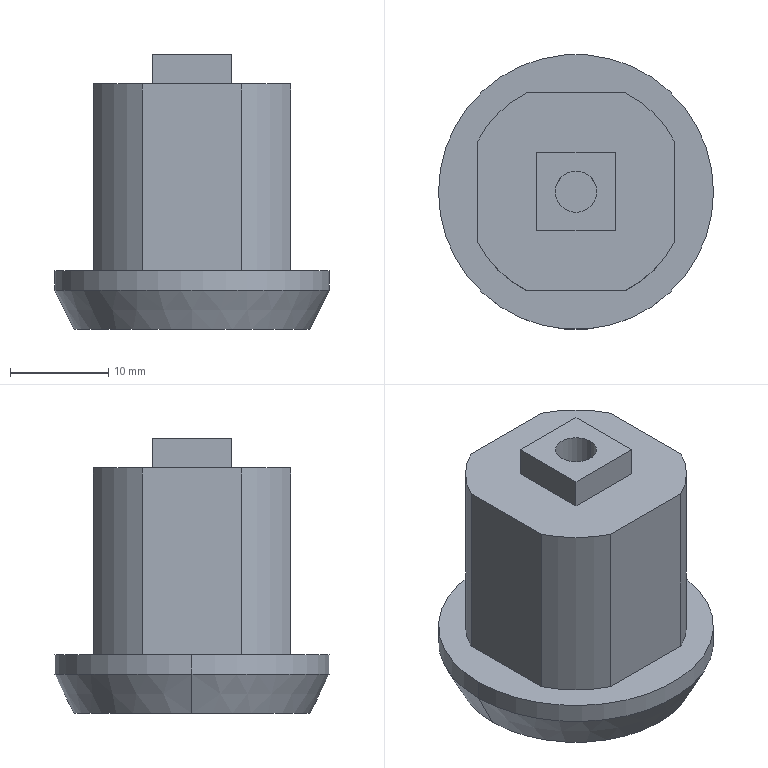Component | SolidWorks | LeftDoorPanelAssembly-1_Lock(MS407)-1 | 1 solid | 32 faces | box 28 x 28 x 28 mm | volume 10078 mm3 | plane 22 | cylinder 8 | cone 2 | commonest cylinder face diameters 22.5 x4 4.2 x2 28 x2
build123d program:
from build123d import *

# Parameters (mm, degrees)
BOSS_EXTRUDE1_DEPTH = 19
SKETCH2_R           = 14
BOSS_EXTRUDE2_DEPTH = 6
CHAMFER1_SIZE       = 4
CHAMFER1_SIZE2      = 2
SKETCH3_W           = 2.8
SKETCH3_H           = 12
CUT_EXTRUDE1_DEPTH  = 10
SKETCH4_W           = 8
SKETCH4_H           = 8
BOSS_EXTRUDE3_DEPTH = 3
SKETCH5_R           = 2.1
CUT_EXTRUDE2_DEPTH  = 5
CHAMFER2_SIZE       = 0.2


with BuildPart() as part:
    # Sketch1 → Boss-Extrude1 (new body)
    with BuildSketch(Plane.XY):
        with BuildLine():
            Line((-10.05, 5.056), (-10.05, -5.056))
            ThreePointArc((-10.05, -5.056), (-7.955, -7.955), (-5.056, -10.05))
            Line((-5.056, -10.05), (5.056, -10.05))
            ThreePointArc((5.056, -10.05), (7.955, -7.955), (10.05, -5.056))
            Line((10.05, -5.056), (10.05, 5.056))
            ThreePointArc((10.05, 5.056), (7.955, 7.955), (5.056, 10.05))
            Line((5.056, 10.05), (-5.056, 10.05))
            ThreePointArc((-5.056, 10.05), (-7.955, 7.955), (-10.05, 5.056))
        make_face()
    extrude(amount=BOSS_EXTRUDE1_DEPTH)

    # Sketch2 → Boss-Extrude2 (add)
    with BuildSketch(Plane(origin=(0, 0, 0), x_dir=(-1, 0, 0), z_dir=(0, 0, -1))):
        Circle(SKETCH2_R)
    extrude(amount=BOSS_EXTRUDE2_DEPTH)

    # Chamfer1
    chamfer1_edges = [part.edges().sort_by_distance(p)[0] for p in [
        (14, 0, -6),
    ]]
    chamfer1_side = [part.faces().sort_by_distance(p)[0] for p in [
        (14, 0, -3),
    ]]
    chamfer(chamfer1_edges, length=CHAMFER1_SIZE, length2=CHAMFER1_SIZE2, reference=chamfer1_side[0])

    # Sketch3 → Cut-Extrude1 (cut)
    with BuildSketch(Plane(origin=(0, 0, -6), x_dir=(-1, 0, 0), z_dir=(0, 0, -1))):
        Rectangle(SKETCH3_W, SKETCH3_H)
    extrude(amount=-CUT_EXTRUDE1_DEPTH, mode=Mode.SUBTRACT)

    # Sketch4 → Boss-Extrude3 (add)
    with BuildSketch(Plane.XY.offset(19)):
        Rectangle(SKETCH4_W, SKETCH4_H)
    extrude(amount=BOSS_EXTRUDE3_DEPTH)

    # Sketch5 → Cut-Extrude2 (cut)
    with BuildSketch(Plane.XY.offset(22)):
        Circle(SKETCH5_R)
    extrude(amount=-CUT_EXTRUDE2_DEPTH, mode=Mode.SUBTRACT)

    # Chamfer2
    chamfer2_edges = [part.edges().sort_by_distance(p)[0] for p in [
        (1.4, 0, -6),
        (0, -6, -6),
        (-1.4, 0, -6),
        (0, 6, -6),
    ]]
    chamfer(chamfer2_edges, length=CHAMFER2_SIZE)


solid = part.part

# Placed as in the assembly
solid = solid.moved(Location((0.6118, 13.542, -73.1), (0, 0, 0)))
STEP:
#1=CARTESIAN_POINT('',(-0.05859,0.5331,-2.209));
#2=VERTEX_POINT('',#1);
#3=CARTESIAN_POINT('',(0.1068,0.5331,-2.209));
#4=VERTEX_POINT('',#3);
#5=CARTESIAN_POINT('',(0.02409,0.5331,-2.209));
#6=DIRECTION('',(0.,0.,1.));
#7=DIRECTION('',(1.,0.,0.));
#8=AXIS2_PLACEMENT_3D('',#5,#6,#7);
#9=CIRCLE('',#8,0.08268);
#10=EDGE_CURVE('',#2,#4,#9,.T.);
#11=ORIENTED_EDGE('',*,*,#10,.F.);
#12=CARTESIAN_POINT('',(-0.05859,0.5331,-2.012));
#13=VERTEX_POINT('',#12);
#14=CARTESIAN_POINT('',(-0.05859,0.5331,-2.209));
#15=DIRECTION('',(0.,0.,1.));
#16=VECTOR('',#15,39.37);
#17=LINE('',#14,#16);
#18=EDGE_CURVE('',#2,#13,#17,.T.);
#19=ORIENTED_EDGE('',*,*,#18,.T.);
#20=CARTESIAN_POINT('',(0.1068,0.5331,-2.012));
#21=VERTEX_POINT('',#20);
#22=CARTESIAN_POINT('',(0.02409,0.5331,-2.012));
#23=DIRECTION('',(0.,0.,1.));
#24=DIRECTION('',(1.,0.,0.));
#25=AXIS2_PLACEMENT_3D('',#22,#23,#24);
#26=CIRCLE('',#25,0.08268);
#27=EDGE_CURVE('',#13,#21,#26,.T.);
#28=ORIENTED_EDGE('',*,*,#27,.T.);
#29=CARTESIAN_POINT('',(0.1068,0.5331,-2.209));
#30=DIRECTION('',(0.,0.,1.));
#31=VECTOR('',#30,39.37);
#32=LINE('',#29,#31);
#33=EDGE_CURVE('',#4,#21,#32,.T.);
#34=ORIENTED_EDGE('',*,*,#33,.F.);
#35=EDGE_LOOP('',(#11,#19,#28,#34));
#36=FACE_OUTER_BOUND('',#35,.T.);
#37=CARTESIAN_POINT('',(0.02409,0.5331,-2.209));
#38=DIRECTION('',(0.,0.,1.));
#39=DIRECTION('',(1.,0.,0.));
#40=AXIS2_PLACEMENT_3D('',#37,#38,#39);
#41=CYLINDRICAL_SURFACE('',#40,0.08268);
#42=ADVANCED_FACE('',(#36),#41,.F.);
#43=CARTESIAN_POINT('',(-0.4484,0.5331,-3.114));
#44=VERTEX_POINT('',#43);
#45=CARTESIAN_POINT('',(0.4965,0.5331,-3.114));
#46=VERTEX_POINT('',#45);
#47=CARTESIAN_POINT('',(0.02409,0.5331,-3.114));
#48=DIRECTION('',(0.,0.,-1.));
#49=DIRECTION('',(-1.,0.,0.));
#50=AXIS2_PLACEMENT_3D('',#47,#48,#49);
#51=CIRCLE('',#50,0.4724);
#52=EDGE_CURVE('',#44,#46,#51,.T.);
#53=ORIENTED_EDGE('',*,*,#52,.F.);
#54=CARTESIAN_POINT('',(-0.5271,0.5331,-2.957));
#55=VERTEX_POINT('',#54);
#56=CARTESIAN_POINT('',(-0.4484,0.5331,-3.114));
#57=DIRECTION('',(-0.4472,0.,0.8944));
#58=VECTOR('',#57,39.37);
#59=LINE('',#56,#58);
#60=EDGE_CURVE('',#44,#55,#59,.T.);
#61=ORIENTED_EDGE('',*,*,#60,.T.);
#62=CARTESIAN_POINT('',(0.5753,0.5331,-2.957));
#63=VERTEX_POINT('',#62);
#64=CARTESIAN_POINT('',(0.02409,0.5331,-2.957));
#65=DIRECTION('',(0.,0.,1.));
#66=DIRECTION('',(-1.,0.,0.));
#67=AXIS2_PLACEMENT_3D('',#64,#65,#66);
#68=CIRCLE('',#67,0.5512);
#69=EDGE_CURVE('',#63,#55,#68,.T.);
#70=ORIENTED_EDGE('',*,*,#69,.F.);
#71=CARTESIAN_POINT('',(0.4965,0.5331,-3.114));
#72=DIRECTION('',(0.4472,0.,0.8944));
#73=VECTOR('',#72,39.37);
#74=LINE('',#71,#73);
#75=EDGE_CURVE('',#46,#63,#74,.T.);
#76=ORIENTED_EDGE('',*,*,#75,.F.);
#77=EDGE_LOOP('',(#53,#61,#70,#76));
#78=FACE_OUTER_BOUND('',#77,.T.);
#79=CARTESIAN_POINT('',(0.02409,0.5331,-3.114));
#80=DIRECTION('',(0.,0.,1.));
#81=DIRECTION('',(1.,0.,0.));
#82=AXIS2_PLACEMENT_3D('',#79,#80,#81);
#83=CONICAL_SURFACE('',#82,0.4724,0.4636);
#84=ADVANCED_FACE('',(#78),#83,.T.);
#85=ORIENTED_EDGE('',*,*,#69,.T.);
#86=CARTESIAN_POINT('',(-0.5271,0.5331,-2.878));
#87=VERTEX_POINT('',#86);
#88=CARTESIAN_POINT('',(-0.5271,0.5331,-3.114));
#89=DIRECTION('',(0.,0.,1.));
#90=VECTOR('',#89,39.37);
#91=LINE('',#88,#90);
#92=EDGE_CURVE('',#55,#87,#91,.T.);
#93=ORIENTED_EDGE('',*,*,#92,.T.);
#94=CARTESIAN_POINT('',(0.5753,0.5331,-2.878));
#95=VERTEX_POINT('',#94);
#96=CARTESIAN_POINT('',(0.02409,0.5331,-2.878));
#97=DIRECTION('',(0.,0.,-1.));
#98=DIRECTION('',(-1.,0.,0.));
#99=AXIS2_PLACEMENT_3D('',#96,#97,#98);
#100=CIRCLE('',#99,0.5512);
#101=EDGE_CURVE('',#87,#95,#100,.T.);
#102=ORIENTED_EDGE('',*,*,#101,.T.);
#103=CARTESIAN_POINT('',(0.5753,0.5331,-3.114));
#104=DIRECTION('',(0.,0.,1.));
#105=VECTOR('',#104,39.37);
#106=LINE('',#103,#105);
#107=EDGE_CURVE('',#63,#95,#106,.T.);
#108=ORIENTED_EDGE('',*,*,#107,.F.);
#109=EDGE_LOOP('',(#85,#93,#102,#108));
#110=FACE_OUTER_BOUND('',#109,.T.);
#111=CARTESIAN_POINT('',(0.02409,0.5331,-3.114));
#112=DIRECTION('',(0.,0.,1.));
#113=DIRECTION('',(1.,0.,0.));
#114=AXIS2_PLACEMENT_3D('',#111,#112,#113);
#115=CYLINDRICAL_SURFACE('',#114,0.5512);
#116=ADVANCED_FACE('',(#110),#115,.T.);
#117=CARTESIAN_POINT('',(-0.175,0.9288,-2.13));
#118=VERTEX_POINT('',#117);
#119=CARTESIAN_POINT('',(-0.3716,0.7322,-2.13));
#120=VERTEX_POINT('',#119);
#121=CARTESIAN_POINT('',(0.02409,0.5331,-2.13));
#122=DIRECTION('',(0.,0.,1.));
#123=DIRECTION('',(1.,0.,0.));
#124=AXIS2_PLACEMENT_3D('',#121,#122,#123);
#125=CIRCLE('',#124,0.4429);
#126=EDGE_CURVE('',#118,#120,#125,.T.);
#127=ORIENTED_EDGE('',*,*,#126,.T.);
#128=CARTESIAN_POINT('',(-0.3716,0.3341,-2.13));
#129=VERTEX_POINT('',#128);
#130=CARTESIAN_POINT('',(-0.3716,0.7322,-2.13));
#131=DIRECTION('',(0.,-1.,0.));
#132=VECTOR('',#131,39.37);
#133=LINE('',#130,#132);
#134=EDGE_CURVE('',#120,#129,#133,.T.);
#135=ORIENTED_EDGE('',*,*,#134,.T.);
#136=CARTESIAN_POINT('',(-0.175,0.1375,-2.13));
#137=VERTEX_POINT('',#136);
#138=CARTESIAN_POINT('',(0.02409,0.5331,-2.13));
#139=DIRECTION('',(0.,0.,1.));
#140=DIRECTION('',(1.,0.,0.));
#141=AXIS2_PLACEMENT_3D('',#138,#139,#140);
#142=CIRCLE('',#141,0.4429);
#143=EDGE_CURVE('',#129,#137,#142,.T.);
#144=ORIENTED_EDGE('',*,*,#143,.T.);
#145=CARTESIAN_POINT('',(0.2231,0.1375,-2.13));
#146=VERTEX_POINT('',#145);
#147=CARTESIAN_POINT('',(-0.175,0.1375,-2.13));
#148=DIRECTION('',(1.,0.,0.));
#149=VECTOR('',#148,39.37);
#150=LINE('',#147,#149);
#151=EDGE_CURVE('',#137,#146,#150,.T.);
#152=ORIENTED_EDGE('',*,*,#151,.T.);
#153=CARTESIAN_POINT('',(0.4198,0.3341,-2.13));
#154=VERTEX_POINT('',#153);
#155=CARTESIAN_POINT('',(0.02409,0.5331,-2.13));
#156=DIRECTION('',(0.,0.,1.));
#157=DIRECTION('',(1.,0.,0.));
#158=AXIS2_PLACEMENT_3D('',#155,#156,#157);
#159=CIRCLE('',#158,0.4429);
#160=EDGE_CURVE('',#146,#154,#159,.T.);
#161=ORIENTED_EDGE('',*,*,#160,.T.);
#162=CARTESIAN_POINT('',(0.4198,0.7322,-2.13));
#163=VERTEX_POINT('',#162);
#164=CARTESIAN_POINT('',(0.4198,0.3341,-2.13));
#165=DIRECTION('',(0.,1.,0.));
#166=VECTOR('',#165,39.37);
#167=LINE('',#164,#166);
#168=EDGE_CURVE('',#154,#163,#167,.T.);
#169=ORIENTED_EDGE('',*,*,#168,.T.);
#170=CARTESIAN_POINT('',(0.2231,0.9288,-2.13));
#171=VERTEX_POINT('',#170);
#172=CARTESIAN_POINT('',(0.02409,0.5331,-2.13));
#173=DIRECTION('',(0.,0.,1.));
#174=DIRECTION('',(1.,0.,0.));
#175=AXIS2_PLACEMENT_3D('',#172,#173,#174);
#176=CIRCLE('',#175,0.4429);
#177=EDGE_CURVE('',#163,#171,#176,.T.);
#178=ORIENTED_EDGE('',*,*,#177,.T.);
#179=CARTESIAN_POINT('',(0.2231,0.9288,-2.13));
#180=DIRECTION('',(-1.,0.,0.));
#181=VECTOR('',#180,39.37);
#182=LINE('',#179,#181);
#183=EDGE_CURVE('',#171,#118,#182,.T.);
#184=ORIENTED_EDGE('',*,*,#183,.T.);
#185=EDGE_LOOP('',(#127,#135,#144,#152,#161,#169,#178,#184));
#186=FACE_OUTER_BOUND('',#185,.T.);
#187=CARTESIAN_POINT('',(-0.1334,0.3757,-2.13));
#188=VERTEX_POINT('',#187);
#189=CARTESIAN_POINT('',(0.1816,0.3757,-2.13));
#190=VERTEX_POINT('',#189);
#191=CARTESIAN_POINT('',(0.1816,0.3757,-2.13));
#192=DIRECTION('',(1.,0.,0.));
#193=VECTOR('',#192,39.37);
#194=LINE('',#191,#193);
#195=EDGE_CURVE('',#188,#190,#194,.T.);
#196=ORIENTED_EDGE('',*,*,#195,.F.);
#197=CARTESIAN_POINT('',(-0.1334,0.6906,-2.13));
#198=VERTEX_POINT('',#197);
#199=CARTESIAN_POINT('',(-0.1334,0.3757,-2.13));
#200=DIRECTION('',(0.,-1.,0.));
#201=VECTOR('',#200,39.37);
#202=LINE('',#199,#201);
#203=EDGE_CURVE('',#198,#188,#202,.T.);
#204=ORIENTED_EDGE('',*,*,#203,.F.);
#205=CARTESIAN_POINT('',(0.1816,0.6906,-2.13));
#206=VERTEX_POINT('',#205);
#207=CARTESIAN_POINT('',(0.1816,0.6906,-2.13));
#208=DIRECTION('',(-1.,-0.,0.));
#209=VECTOR('',#208,39.37);
#210=LINE('',#207,#209);
#211=EDGE_CURVE('',#206,#198,#210,.T.);
#212=ORIENTED_EDGE('',*,*,#211,.F.);
#213=CARTESIAN_POINT('',(0.1816,0.3757,-2.13));
#214=DIRECTION('',(0.,1.,0.));
#215=VECTOR('',#214,39.37);
#216=LINE('',#213,#215);
#217=EDGE_CURVE('',#190,#206,#216,.T.);
#218=ORIENTED_EDGE('',*,*,#217,.F.);
#219=EDGE_LOOP('',(#196,#204,#212,#218));
#220=FACE_BOUND('',#219,.T.);
#221=CARTESIAN_POINT('',(0.02409,0.5331,-2.13));
#222=DIRECTION('',(0.,0.,1.));
#223=DIRECTION('',(1.,0.,0.));
#224=AXIS2_PLACEMENT_3D('',#221,#222,#223);
#225=PLANE('',#224);
#226=ADVANCED_FACE('',(#186,#220),#225,.T.);
#227=CARTESIAN_POINT('',(-0.175,0.9288,-2.878));
#228=VERTEX_POINT('',#227);
#229=CARTESIAN_POINT('',(-0.3716,0.7322,-2.878));
#230=VERTEX_POINT('',#229);
#231=CARTESIAN_POINT('',(0.02409,0.5331,-2.878));
#232=DIRECTION('',(0.,0.,1.));
#233=DIRECTION('',(1.,0.,0.));
#234=AXIS2_PLACEMENT_3D('',#231,#232,#233);
#235=CIRCLE('',#234,0.4429);
#236=EDGE_CURVE('',#228,#230,#235,.T.);
#237=ORIENTED_EDGE('',*,*,#236,.T.);
#238=CARTESIAN_POINT('',(-0.3716,0.7322,-2.13));
#239=DIRECTION('',(0.,0.,-1.));
#240=VECTOR('',#239,39.37);
#241=LINE('',#238,#240);
#242=EDGE_CURVE('',#120,#230,#241,.T.);
#243=ORIENTED_EDGE('',*,*,#242,.F.);
#244=ORIENTED_EDGE('',*,*,#126,.F.);
#245=CARTESIAN_POINT('',(-0.175,0.9288,-2.13));
#246=DIRECTION('',(0.,0.,-1.));
#247=VECTOR('',#246,39.37);
#248=LINE('',#245,#247);
#249=EDGE_CURVE('',#118,#228,#248,.T.);
#250=ORIENTED_EDGE('',*,*,#249,.T.);
#251=EDGE_LOOP('',(#237,#243,#244,#250));
#252=FACE_OUTER_BOUND('',#251,.T.);
#253=CARTESIAN_POINT('',(0.02409,0.5331,-2.13));
#254=DIRECTION('',(0.,0.,-1.));
#255=DIRECTION('',(-1.,0.,0.));
#256=AXIS2_PLACEMENT_3D('',#253,#254,#255);
#257=CYLINDRICAL_SURFACE('',#256,0.4429);
#258=ADVANCED_FACE('',(#252),#257,.T.);
#259=CARTESIAN_POINT('',(-0.3716,0.3341,-2.878));
#260=VERTEX_POINT('',#259);
#261=CARTESIAN_POINT('',(-0.3716,0.7322,-2.878));
#262=DIRECTION('',(0.,-1.,0.));
#263=VECTOR('',#262,39.37);
#264=LINE('',#261,#263);
#265=EDGE_CURVE('',#230,#260,#264,.T.);
#266=ORIENTED_EDGE('',*,*,#265,.T.);
#267=CARTESIAN_POINT('',(-0.3716,0.3341,-2.13));
#268=DIRECTION('',(0.,0.,-1.));
#269=VECTOR('',#268,39.37);
#270=LINE('',#267,#269);
#271=EDGE_CURVE('',#129,#260,#270,.T.);
#272=ORIENTED_EDGE('',*,*,#271,.F.);
#273=ORIENTED_EDGE('',*,*,#134,.F.);
#274=ORIENTED_EDGE('',*,*,#242,.T.);
#275=EDGE_LOOP('',(#266,#272,#273,#274));
#276=FACE_OUTER_BOUND('',#275,.T.);
#277=CARTESIAN_POINT('',(-0.3716,0.7322,-2.13));
#278=DIRECTION('',(1.,0.,0.));
#279=DIRECTION('',(0.,0.,-1.));
#280=AXIS2_PLACEMENT_3D('',#277,#278,#279);
#281=PLANE('',#280);
#282=ADVANCED_FACE('',(#276),#281,.F.);
#283=CARTESIAN_POINT('',(-0.175,0.1375,-2.878));
#284=VERTEX_POINT('',#283);
#285=CARTESIAN_POINT('',(0.02409,0.5331,-2.878));
#286=DIRECTION('',(0.,0.,1.));
#287=DIRECTION('',(1.,0.,0.));
#288=AXIS2_PLACEMENT_3D('',#285,#286,#287);
#289=CIRCLE('',#288,0.4429);
#290=EDGE_CURVE('',#260,#284,#289,.T.);
#291=ORIENTED_EDGE('',*,*,#290,.T.);
#292=CARTESIAN_POINT('',(-0.175,0.1375,-2.13));
#293=DIRECTION('',(0.,0.,-1.));
#294=VECTOR('',#293,39.37);
#295=LINE('',#292,#294);
#296=EDGE_CURVE('',#137,#284,#295,.T.);
#297=ORIENTED_EDGE('',*,*,#296,.F.);
#298=ORIENTED_EDGE('',*,*,#143,.F.);
#299=ORIENTED_EDGE('',*,*,#271,.T.);
#300=EDGE_LOOP('',(#291,#297,#298,#299));
#301=FACE_OUTER_BOUND('',#300,.T.);
#302=CARTESIAN_POINT('',(0.02409,0.5331,-2.13));
#303=DIRECTION('',(0.,0.,-1.));
#304=DIRECTION('',(-1.,0.,0.));
#305=AXIS2_PLACEMENT_3D('',#302,#303,#304);
#306=CYLINDRICAL_SURFACE('',#305,0.4429);
#307=ADVANCED_FACE('',(#301),#306,.T.);
#308=CARTESIAN_POINT('',(0.2231,0.1375,-2.878));
#309=VERTEX_POINT('',#308);
#310=CARTESIAN_POINT('',(-0.175,0.1375,-2.878));
#311=DIRECTION('',(1.,0.,0.));
#312=VECTOR('',#311,39.37);
#313=LINE('',#310,#312);
#314=EDGE_CURVE('',#284,#309,#313,.T.);
#315=ORIENTED_EDGE('',*,*,#314,.T.);
#316=CARTESIAN_POINT('',(0.2231,0.1375,-2.13));
#317=DIRECTION('',(0.,0.,-1.));
#318=VECTOR('',#317,39.37);
#319=LINE('',#316,#318);
#320=EDGE_CURVE('',#146,#309,#319,.T.);
#321=ORIENTED_EDGE('',*,*,#320,.F.);
#322=ORIENTED_EDGE('',*,*,#151,.F.);
#323=ORIENTED_EDGE('',*,*,#296,.T.);
#324=EDGE_LOOP('',(#315,#321,#322,#323));
#325=FACE_OUTER_BOUND('',#324,.T.);
#326=CARTESIAN_POINT('',(-0.175,0.1375,-2.13));
#327=DIRECTION('',(0.,1.,0.));
#328=DIRECTION('',(0.,0.,1.));
#329=AXIS2_PLACEMENT_3D('',#326,#327,#328);
#330=PLANE('',#329);
#331=ADVANCED_FACE('',(#325),#330,.F.);
#332=CARTESIAN_POINT('',(0.4198,0.3341,-2.878));
#333=VERTEX_POINT('',#332);
#334=CARTESIAN_POINT('',(0.02409,0.5331,-2.878));
#335=DIRECTION('',(0.,0.,1.));
#336=DIRECTION('',(1.,0.,0.));
#337=AXIS2_PLACEMENT_3D('',#334,#335,#336);
#338=CIRCLE('',#337,0.4429);
#339=EDGE_CURVE('',#309,#333,#338,.T.);
#340=ORIENTED_EDGE('',*,*,#339,.T.);
#341=CARTESIAN_POINT('',(0.4198,0.3341,-2.13));
#342=DIRECTION('',(0.,0.,-1.));
#343=VECTOR('',#342,39.37);
#344=LINE('',#341,#343);
#345=EDGE_CURVE('',#154,#333,#344,.T.);
#346=ORIENTED_EDGE('',*,*,#345,.F.);
#347=ORIENTED_EDGE('',*,*,#160,.F.);
#348=ORIENTED_EDGE('',*,*,#320,.T.);
#349=EDGE_LOOP('',(#340,#346,#347,#348));
#350=FACE_OUTER_BOUND('',#349,.T.);
#351=CARTESIAN_POINT('',(0.02409,0.5331,-2.13));
#352=DIRECTION('',(0.,0.,-1.));
#353=DIRECTION('',(-1.,0.,0.));
#354=AXIS2_PLACEMENT_3D('',#351,#352,#353);
#355=CYLINDRICAL_SURFACE('',#354,0.4429);
#356=ADVANCED_FACE('',(#350),#355,.T.);
#357=CARTESIAN_POINT('',(0.4198,0.7322,-2.878));
#358=VERTEX_POINT('',#357);
#359=CARTESIAN_POINT('',(0.4198,0.3341,-2.878));
#360=DIRECTION('',(0.,1.,0.));
#361=VECTOR('',#360,39.37);
#362=LINE('',#359,#361);
#363=EDGE_CURVE('',#333,#358,#362,.T.);
#364=ORIENTED_EDGE('',*,*,#363,.T.);
#365=CARTESIAN_POINT('',(0.4198,0.7322,-2.13));
#366=DIRECTION('',(0.,0.,-1.));
#367=VECTOR('',#366,39.37);
#368=LINE('',#365,#367);
#369=EDGE_CURVE('',#163,#358,#368,.T.);
#370=ORIENTED_EDGE('',*,*,#369,.F.);
#371=ORIENTED_EDGE('',*,*,#168,.F.);
#372=ORIENTED_EDGE('',*,*,#345,.T.);
#373=EDGE_LOOP('',(#364,#370,#371,#372));
#374=FACE_OUTER_BOUND('',#373,.T.);
#375=CARTESIAN_POINT('',(0.4198,0.3341,-2.13));
#376=DIRECTION('',(-1.,0.,0.));
#377=DIRECTION('',(-0.,-1.,0.));
#378=AXIS2_PLACEMENT_3D('',#375,#376,#377);
#379=PLANE('',#378);
#380=ADVANCED_FACE('',(#374),#379,.F.);
#381=CARTESIAN_POINT('',(0.2231,0.9288,-2.878));
#382=VERTEX_POINT('',#381);
#383=CARTESIAN_POINT('',(0.02409,0.5331,-2.878));
#384=DIRECTION('',(0.,0.,1.));
#385=DIRECTION('',(1.,0.,0.));
#386=AXIS2_PLACEMENT_3D('',#383,#384,#385);
#387=CIRCLE('',#386,0.4429);
#388=EDGE_CURVE('',#358,#382,#387,.T.);
#389=ORIENTED_EDGE('',*,*,#388,.T.);
#390=CARTESIAN_POINT('',(0.2231,0.9288,-2.13));
#391=DIRECTION('',(0.,0.,-1.));
#392=VECTOR('',#391,39.37);
#393=LINE('',#390,#392);
#394=EDGE_CURVE('',#171,#382,#393,.T.);
#395=ORIENTED_EDGE('',*,*,#394,.F.);
#396=ORIENTED_EDGE('',*,*,#177,.F.);
#397=ORIENTED_EDGE('',*,*,#369,.T.);
#398=EDGE_LOOP('',(#389,#395,#396,#397));
#399=FACE_OUTER_BOUND('',#398,.T.);
#400=CARTESIAN_POINT('',(0.02409,0.5331,-2.13));
#401=DIRECTION('',(0.,0.,-1.));
#402=DIRECTION('',(-1.,0.,0.));
#403=AXIS2_PLACEMENT_3D('',#400,#401,#402);
#404=CYLINDRICAL_SURFACE('',#403,0.4429);
#405=ADVANCED_FACE('',(#399),#404,.T.);
#406=CARTESIAN_POINT('',(0.2231,0.9288,-2.878));
#407=DIRECTION('',(-1.,0.,0.));
#408=VECTOR('',#407,39.37);
#409=LINE('',#406,#408);
#410=EDGE_CURVE('',#382,#228,#409,.T.);
#411=ORIENTED_EDGE('',*,*,#410,.T.);
#412=ORIENTED_EDGE('',*,*,#249,.F.);
#413=ORIENTED_EDGE('',*,*,#183,.F.);
#414=ORIENTED_EDGE('',*,*,#394,.T.);
#415=EDGE_LOOP('',(#411,#412,#413,#414));
#416=FACE_OUTER_BOUND('',#415,.T.);
#417=CARTESIAN_POINT('',(0.2231,0.9288,-2.13));
#418=DIRECTION('',(0.,-1.,0.));
#419=DIRECTION('',(0.,0.,-1.));
#420=AXIS2_PLACEMENT_3D('',#417,#418,#419);
#421=PLANE('',#420);
#422=ADVANCED_FACE('',(#416),#421,.F.);
#423=CARTESIAN_POINT('',(0.02409,0.5331,-2.878));
#424=DIRECTION('',(0.,0.,-1.));
#425=DIRECTION('',(-1.,0.,0.));
#426=AXIS2_PLACEMENT_3D('',#423,#424,#425);
#427=CIRCLE('',#426,0.5512);
#428=EDGE_CURVE('',#95,#87,#427,.T.);
#429=ORIENTED_EDGE('',*,*,#428,.F.);
#430=ORIENTED_EDGE('',*,*,#101,.F.);
#431=EDGE_LOOP('',(#429,#430));
#432=FACE_OUTER_BOUND('',#431,.T.);
#433=ORIENTED_EDGE('',*,*,#265,.F.);
#434=ORIENTED_EDGE('',*,*,#236,.F.);
#435=ORIENTED_EDGE('',*,*,#410,.F.);
#436=ORIENTED_EDGE('',*,*,#388,.F.);
#437=ORIENTED_EDGE('',*,*,#363,.F.);
#438=ORIENTED_EDGE('',*,*,#339,.F.);
#439=ORIENTED_EDGE('',*,*,#314,.F.);
#440=ORIENTED_EDGE('',*,*,#290,.F.);
#441=EDGE_LOOP('',(#433,#434,#435,#436,#437,#438,#439,#440));
#442=FACE_BOUND('',#441,.T.);
#443=CARTESIAN_POINT('',(0.02409,0.5331,-2.878));
#444=DIRECTION('',(0.,0.,-1.));
#445=DIRECTION('',(-1.,0.,0.));
#446=AXIS2_PLACEMENT_3D('',#443,#444,#445);
#447=PLANE('',#446);
#448=ADVANCED_FACE('',(#432,#442),#447,.F.);
#449=ORIENTED_EDGE('',*,*,#92,.F.);
#450=CARTESIAN_POINT('',(0.02409,0.5331,-2.957));
#451=DIRECTION('',(0.,0.,1.));
#452=DIRECTION('',(-1.,0.,0.));
#453=AXIS2_PLACEMENT_3D('',#450,#451,#452);
#454=CIRCLE('',#453,0.5512);
#455=EDGE_CURVE('',#55,#63,#454,.T.);
#456=ORIENTED_EDGE('',*,*,#455,.T.);
#457=ORIENTED_EDGE('',*,*,#107,.T.);
#458=ORIENTED_EDGE('',*,*,#428,.T.);
#459=EDGE_LOOP('',(#449,#456,#457,#458));
#460=FACE_OUTER_BOUND('',#459,.T.);
#461=CARTESIAN_POINT('',(0.02409,0.5331,-3.114));
#462=DIRECTION('',(0.,0.,1.));
#463=DIRECTION('',(1.,0.,0.));
#464=AXIS2_PLACEMENT_3D('',#461,#462,#463);
#465=CYLINDRICAL_SURFACE('',#464,0.5512);
#466=ADVANCED_FACE('',(#460),#465,.T.);
#467=CARTESIAN_POINT('',(-0.03891,0.289,-3.114));
#468=VERTEX_POINT('',#467);
#469=CARTESIAN_POINT('',(0.08708,0.289,-3.114));
#470=VERTEX_POINT('',#469);
#471=CARTESIAN_POINT('',(0.0792,0.289,-3.114));
#472=DIRECTION('',(1.,0.,0.));
#473=VECTOR('',#472,39.37);
#474=LINE('',#471,#473);
#475=EDGE_CURVE('',#468,#470,#474,.T.);
#476=ORIENTED_EDGE('',*,*,#475,.T.);
#477=CARTESIAN_POINT('',(0.08708,0.7772,-3.114));
#478=VERTEX_POINT('',#477);
#479=CARTESIAN_POINT('',(0.08708,0.7694,-3.114));
#480=DIRECTION('',(0.,1.,0.));
#481=VECTOR('',#480,39.37);
#482=LINE('',#479,#481);
#483=EDGE_CURVE('',#470,#478,#482,.T.);
#484=ORIENTED_EDGE('',*,*,#483,.T.);
#485=CARTESIAN_POINT('',(-0.03891,0.7772,-3.114));
#486=VERTEX_POINT('',#485);
#487=CARTESIAN_POINT('',(-0.03103,0.7772,-3.114));
#488=DIRECTION('',(-1.,0.,0.));
#489=VECTOR('',#488,39.37);
#490=LINE('',#487,#489);
#491=EDGE_CURVE('',#478,#486,#490,.T.);
#492=ORIENTED_EDGE('',*,*,#491,.T.);
#493=CARTESIAN_POINT('',(-0.03891,0.2969,-3.114));
#494=DIRECTION('',(0.,-1.,0.));
#495=VECTOR('',#494,39.37);
#496=LINE('',#493,#495);
#497=EDGE_CURVE('',#486,#468,#496,.T.);
#498=ORIENTED_EDGE('',*,*,#497,.T.);
#499=EDGE_LOOP('',(#476,#484,#492,#498));
#500=FACE_BOUND('',#499,.T.);
#501=CARTESIAN_POINT('',(0.02409,0.5331,-3.114));
#502=DIRECTION('',(0.,0.,-1.));
#503=DIRECTION('',(-1.,0.,0.));
#504=AXIS2_PLACEMENT_3D('',#501,#502,#503);
#505=CIRCLE('',#504,0.4724);
#506=EDGE_CURVE('',#46,#44,#505,.T.);
#507=ORIENTED_EDGE('',*,*,#506,.T.);
#508=ORIENTED_EDGE('',*,*,#52,.T.);
#509=EDGE_LOOP('',(#507,#508));
#510=FACE_OUTER_BOUND('',#509,.T.);
#511=CARTESIAN_POINT('',(0.02409,0.5331,-3.114));
#512=DIRECTION('',(0.,0.,-1.));
#513=DIRECTION('',(-1.,0.,0.));
#514=AXIS2_PLACEMENT_3D('',#511,#512,#513);
#515=PLANE('',#514);
#516=ADVANCED_FACE('',(#500,#510),#515,.T.);
#517=ORIENTED_EDGE('',*,*,#60,.F.);
#518=ORIENTED_EDGE('',*,*,#506,.F.);
#519=ORIENTED_EDGE('',*,*,#75,.T.);
#520=ORIENTED_EDGE('',*,*,#455,.F.);
#521=EDGE_LOOP('',(#517,#518,#519,#520));
#522=FACE_OUTER_BOUND('',#521,.T.);
#523=CARTESIAN_POINT('',(0.02409,0.5331,-3.114));
#524=DIRECTION('',(0.,0.,1.));
#525=DIRECTION('',(1.,0.,0.));
#526=AXIS2_PLACEMENT_3D('',#523,#524,#525);
#527=CONICAL_SURFACE('',#526,0.4724,0.4636);
#528=ADVANCED_FACE('',(#522),#527,.T.);
#529=CARTESIAN_POINT('',(0.0792,0.7694,-2.72));
#530=VERTEX_POINT('',#529);
#531=CARTESIAN_POINT('',(0.0792,0.7694,-3.106));
#532=VERTEX_POINT('',#531);
#533=CARTESIAN_POINT('',(0.0792,0.7694,-2.72));
#534=DIRECTION('',(0.,0.,-1.));
#535=VECTOR('',#534,39.37);
#536=LINE('',#533,#535);
#537=EDGE_CURVE('',#530,#532,#536,.T.);
#538=ORIENTED_EDGE('',*,*,#537,.T.);
#539=CARTESIAN_POINT('',(0.0792,0.2969,-3.106));
#540=VERTEX_POINT('',#539);
#541=CARTESIAN_POINT('',(0.0792,0.2969,-3.106));
#542=DIRECTION('',(0.,-1.,0.));
#543=VECTOR('',#542,39.37);
#544=LINE('',#541,#543);
#545=EDGE_CURVE('',#532,#540,#544,.T.);
#546=ORIENTED_EDGE('',*,*,#545,.T.);
#547=CARTESIAN_POINT('',(0.0792,0.2969,-2.72));
#548=VERTEX_POINT('',#547);
#549=CARTESIAN_POINT('',(0.0792,0.2969,-2.72));
#550=DIRECTION('',(0.,0.,-1.));
#551=VECTOR('',#550,39.37);
#552=LINE('',#549,#551);
#553=EDGE_CURVE('',#548,#540,#552,.T.);
#554=ORIENTED_EDGE('',*,*,#553,.F.);
#555=CARTESIAN_POINT('',(0.0792,0.2969,-2.72));
#556=DIRECTION('',(0.,-1.,0.));
#557=VECTOR('',#556,39.37);
#558=LINE('',#555,#557);
#559=EDGE_CURVE('',#530,#548,#558,.T.);
#560=ORIENTED_EDGE('',*,*,#559,.F.);
#561=EDGE_LOOP('',(#538,#546,#554,#560));
#562=FACE_OUTER_BOUND('',#561,.T.);
#563=CARTESIAN_POINT('',(0.0792,0.2969,-2.72));
#564=DIRECTION('',(1.,0.,0.));
#565=DIRECTION('',(0.,0.,-1.));
#566=AXIS2_PLACEMENT_3D('',#563,#564,#565);
#567=PLANE('',#566);
#568=ADVANCED_FACE('',(#562),#567,.F.);
#569=CARTESIAN_POINT('',(-0.03103,0.7694,-2.72));
#570=VERTEX_POINT('',#569);
#571=CARTESIAN_POINT('',(-0.03103,0.7694,-3.106));
#572=VERTEX_POINT('',#571);
#573=CARTESIAN_POINT('',(-0.03103,0.7694,-2.72));
#574=DIRECTION('',(0.,0.,-1.));
#575=VECTOR('',#574,39.37);
#576=LINE('',#573,#575);
#577=EDGE_CURVE('',#570,#572,#576,.T.);
#578=ORIENTED_EDGE('',*,*,#577,.T.);
#579=CARTESIAN_POINT('',(0.0792,0.7694,-3.106));
#580=DIRECTION('',(1.,0.,0.));
#581=VECTOR('',#580,39.37);
#582=LINE('',#579,#581);
#583=EDGE_CURVE('',#572,#532,#582,.T.);
#584=ORIENTED_EDGE('',*,*,#583,.T.);
#585=ORIENTED_EDGE('',*,*,#537,.F.);
#586=CARTESIAN_POINT('',(-0.03103,0.7694,-2.72));
#587=DIRECTION('',(1.,0.,0.));
#588=VECTOR('',#587,39.37);
#589=LINE('',#586,#588);
#590=EDGE_CURVE('',#570,#530,#589,.T.);
#591=ORIENTED_EDGE('',*,*,#590,.F.);
#592=EDGE_LOOP('',(#578,#584,#585,#591));
#593=FACE_OUTER_BOUND('',#592,.T.);
#594=CARTESIAN_POINT('',(-0.03103,0.7694,-2.72));
#595=DIRECTION('',(0.,1.,0.));
#596=DIRECTION('',(0.,0.,1.));
#597=AXIS2_PLACEMENT_3D('',#594,#595,#596);
#598=PLANE('',#597);
#599=ADVANCED_FACE('',(#593),#598,.F.);
#600=CARTESIAN_POINT('',(-0.03103,0.2969,-2.72));
#601=VERTEX_POINT('',#600);
#602=CARTESIAN_POINT('',(-0.03103,0.2969,-3.106));
#603=VERTEX_POINT('',#602);
#604=CARTESIAN_POINT('',(-0.03103,0.2969,-2.72));
#605=DIRECTION('',(0.,0.,-1.));
#606=VECTOR('',#605,39.37);
#607=LINE('',#604,#606);
#608=EDGE_CURVE('',#601,#603,#607,.T.);
#609=ORIENTED_EDGE('',*,*,#608,.T.);
#610=CARTESIAN_POINT('',(-0.03103,0.7694,-3.106));
#611=DIRECTION('',(0.,1.,0.));
#612=VECTOR('',#611,39.37);
#613=LINE('',#610,#612);
#614=EDGE_CURVE('',#603,#572,#613,.T.);
#615=ORIENTED_EDGE('',*,*,#614,.T.);
#616=ORIENTED_EDGE('',*,*,#577,.F.);
#617=CARTESIAN_POINT('',(-0.03103,0.2969,-2.72));
#618=DIRECTION('',(0.,1.,0.));
#619=VECTOR('',#618,39.37);
#620=LINE('',#617,#619);
#621=EDGE_CURVE('',#601,#570,#620,.T.);
#622=ORIENTED_EDGE('',*,*,#621,.F.);
#623=EDGE_LOOP('',(#609,#615,#616,#622));
#624=FACE_OUTER_BOUND('',#623,.T.);
#625=CARTESIAN_POINT('',(-0.03103,0.2969,-2.72));
#626=DIRECTION('',(-1.,0.,0.));
#627=DIRECTION('',(0.,0.,1.));
#628=AXIS2_PLACEMENT_3D('',#625,#626,#627);
#629=PLANE('',#628);
#630=ADVANCED_FACE('',(#624),#629,.F.);
#631=ORIENTED_EDGE('',*,*,#553,.T.);
#632=CARTESIAN_POINT('',(-0.03103,0.2969,-3.106));
#633=DIRECTION('',(-1.,0.,0.));
#634=VECTOR('',#633,39.37);
#635=LINE('',#632,#634);
#636=EDGE_CURVE('',#540,#603,#635,.T.);
#637=ORIENTED_EDGE('',*,*,#636,.T.);
#638=ORIENTED_EDGE('',*,*,#608,.F.);
#639=CARTESIAN_POINT('',(-0.03103,0.2969,-2.72));
#640=DIRECTION('',(-1.,0.,0.));
#641=VECTOR('',#640,39.37);
#642=LINE('',#639,#641);
#643=EDGE_CURVE('',#548,#601,#642,.T.);
#644=ORIENTED_EDGE('',*,*,#643,.F.);
#645=EDGE_LOOP('',(#631,#637,#638,#644));
#646=FACE_OUTER_BOUND('',#645,.T.);
#647=CARTESIAN_POINT('',(-0.03103,0.2969,-2.72));
#648=DIRECTION('',(0.,-1.,0.));
#649=DIRECTION('',(0.,0.,-1.));
#650=AXIS2_PLACEMENT_3D('',#647,#648,#649);
#651=PLANE('',#650);
#652=ADVANCED_FACE('',(#646),#651,.F.);
#653=ORIENTED_EDGE('',*,*,#559,.T.);
#654=ORIENTED_EDGE('',*,*,#643,.T.);
#655=ORIENTED_EDGE('',*,*,#621,.T.);
#656=ORIENTED_EDGE('',*,*,#590,.T.);
#657=EDGE_LOOP('',(#653,#654,#655,#656));
#658=FACE_OUTER_BOUND('',#657,.T.);
#659=CARTESIAN_POINT('',(0.02409,0.5331,-2.72));
#660=DIRECTION('',(0.,0.,-1.));
#661=DIRECTION('',(-1.,0.,0.));
#662=AXIS2_PLACEMENT_3D('',#659,#660,#661);
#663=PLANE('',#662);
#664=ADVANCED_FACE('',(#658),#663,.T.);
#665=ORIENTED_EDGE('',*,*,#203,.T.);
#666=CARTESIAN_POINT('',(-0.1334,0.3757,-2.012));
#667=VERTEX_POINT('',#666);
#668=CARTESIAN_POINT('',(-0.1334,0.3757,-2.012));
#669=DIRECTION('',(0.,0.,-1.));
#670=VECTOR('',#669,39.37);
#671=LINE('',#668,#670);
#672=EDGE_CURVE('',#667,#188,#671,.T.);
#673=ORIENTED_EDGE('',*,*,#672,.F.);
#674=CARTESIAN_POINT('',(-0.1334,0.6906,-2.012));
#675=VERTEX_POINT('',#674);
#676=CARTESIAN_POINT('',(-0.1334,0.3757,-2.012));
#677=DIRECTION('',(0.,-1.,0.));
#678=VECTOR('',#677,39.37);
#679=LINE('',#676,#678);
#680=EDGE_CURVE('',#675,#667,#679,.T.);
#681=ORIENTED_EDGE('',*,*,#680,.F.);
#682=CARTESIAN_POINT('',(-0.1334,0.6906,-2.012));
#683=DIRECTION('',(0.,0.,-1.));
#684=VECTOR('',#683,39.37);
#685=LINE('',#682,#684);
#686=EDGE_CURVE('',#675,#198,#685,.T.);
#687=ORIENTED_EDGE('',*,*,#686,.T.);
#688=EDGE_LOOP('',(#665,#673,#681,#687));
#689=FACE_OUTER_BOUND('',#688,.T.);
#690=CARTESIAN_POINT('',(-0.1334,0.3757,-2.012));
#691=DIRECTION('',(1.,0.,0.));
#692=DIRECTION('',(0.,0.,-1.));
#693=AXIS2_PLACEMENT_3D('',#690,#691,#692);
#694=PLANE('',#693);
#695=ADVANCED_FACE('',(#689),#694,.F.);
#696=ORIENTED_EDGE('',*,*,#195,.T.);
#697=CARTESIAN_POINT('',(0.1816,0.3757,-2.012));
#698=VERTEX_POINT('',#697);
#699=CARTESIAN_POINT('',(0.1816,0.3757,-2.012));
#700=DIRECTION('',(0.,0.,-1.));
#701=VECTOR('',#700,39.37);
#702=LINE('',#699,#701);
#703=EDGE_CURVE('',#698,#190,#702,.T.);
#704=ORIENTED_EDGE('',*,*,#703,.F.);
#705=CARTESIAN_POINT('',(0.1816,0.3757,-2.012));
#706=DIRECTION('',(1.,0.,0.));
#707=VECTOR('',#706,39.37);
#708=LINE('',#705,#707);
#709=EDGE_CURVE('',#667,#698,#708,.T.);
#710=ORIENTED_EDGE('',*,*,#709,.F.);
#711=ORIENTED_EDGE('',*,*,#672,.T.);
#712=EDGE_LOOP('',(#696,#704,#710,#711));
#713=FACE_OUTER_BOUND('',#712,.T.);
#714=CARTESIAN_POINT('',(0.1816,0.3757,-2.012));
#715=DIRECTION('',(-0.,1.,0.));
#716=DIRECTION('',(-1.,-0.,0.));
#717=AXIS2_PLACEMENT_3D('',#714,#715,#716);
#718=PLANE('',#717);
#719=ADVANCED_FACE('',(#713),#718,.F.);
#720=ORIENTED_EDGE('',*,*,#217,.T.);
#721=CARTESIAN_POINT('',(0.1816,0.6906,-2.012));
#722=VERTEX_POINT('',#721);
#723=CARTESIAN_POINT('',(0.1816,0.6906,-2.012));
#724=DIRECTION('',(0.,0.,-1.));
#725=VECTOR('',#724,39.37);
#726=LINE('',#723,#725);
#727=EDGE_CURVE('',#722,#206,#726,.T.);
#728=ORIENTED_EDGE('',*,*,#727,.F.);
#729=CARTESIAN_POINT('',(0.1816,0.3757,-2.012));
#730=DIRECTION('',(0.,1.,0.));
#731=VECTOR('',#730,39.37);
#732=LINE('',#729,#731);
#733=EDGE_CURVE('',#698,#722,#732,.T.);
#734=ORIENTED_EDGE('',*,*,#733,.F.);
#735=ORIENTED_EDGE('',*,*,#703,.T.);
#736=EDGE_LOOP('',(#720,#728,#734,#735));
#737=FACE_OUTER_BOUND('',#736,.T.);
#738=CARTESIAN_POINT('',(0.1816,0.3757,-2.012));
#739=DIRECTION('',(-1.,0.,0.));
#740=DIRECTION('',(0.,0.,1.));
#741=AXIS2_PLACEMENT_3D('',#738,#739,#740);
#742=PLANE('',#741);
#743=ADVANCED_FACE('',(#737),#742,.F.);
#744=ORIENTED_EDGE('',*,*,#211,.T.);
#745=ORIENTED_EDGE('',*,*,#686,.F.);
#746=CARTESIAN_POINT('',(0.1816,0.6906,-2.012));
#747=DIRECTION('',(-1.,-0.,0.));
#748=VECTOR('',#747,39.37);
#749=LINE('',#746,#748);
#750=EDGE_CURVE('',#722,#675,#749,.T.);
#751=ORIENTED_EDGE('',*,*,#750,.F.);
#752=ORIENTED_EDGE('',*,*,#727,.T.);
#753=EDGE_LOOP('',(#744,#745,#751,#752));
#754=FACE_OUTER_BOUND('',#753,.T.);
#755=CARTESIAN_POINT('',(0.1816,0.6906,-2.012));
#756=DIRECTION('',(0.,-1.,0.));
#757=DIRECTION('',(1.,0.,0.));
#758=AXIS2_PLACEMENT_3D('',#755,#756,#757);
#759=PLANE('',#758);
#760=ADVANCED_FACE('',(#754),#759,.F.);
#761=CARTESIAN_POINT('',(0.02409,0.5331,-2.012));
#762=DIRECTION('',(0.,0.,1.));
#763=DIRECTION('',(1.,0.,0.));
#764=AXIS2_PLACEMENT_3D('',#761,#762,#763);
#765=CIRCLE('',#764,0.08268);
#766=EDGE_CURVE('',#21,#13,#765,.T.);
#767=ORIENTED_EDGE('',*,*,#766,.F.);
#768=ORIENTED_EDGE('',*,*,#27,.F.);
#769=EDGE_LOOP('',(#767,#768));
#770=FACE_BOUND('',#769,.T.);
#771=ORIENTED_EDGE('',*,*,#680,.T.);
#772=ORIENTED_EDGE('',*,*,#709,.T.);
#773=ORIENTED_EDGE('',*,*,#733,.T.);
#774=ORIENTED_EDGE('',*,*,#750,.T.);
#775=EDGE_LOOP('',(#771,#772,#773,#774));
#776=FACE_OUTER_BOUND('',#775,.T.);
#777=CARTESIAN_POINT('',(0.02409,0.5331,-2.012));
#778=DIRECTION('',(0.,0.,1.));
#779=DIRECTION('',(1.,0.,0.));
#780=AXIS2_PLACEMENT_3D('',#777,#778,#779);
#781=PLANE('',#780);
#782=ADVANCED_FACE('',(#770,#776),#781,.T.);
#783=ORIENTED_EDGE('',*,*,#18,.F.);
#784=CARTESIAN_POINT('',(0.02409,0.5331,-2.209));
#785=DIRECTION('',(0.,0.,1.));
#786=DIRECTION('',(1.,0.,0.));
#787=AXIS2_PLACEMENT_3D('',#784,#785,#786);
#788=CIRCLE('',#787,0.08268);
#789=EDGE_CURVE('',#4,#2,#788,.T.);
#790=ORIENTED_EDGE('',*,*,#789,.F.);
#791=ORIENTED_EDGE('',*,*,#33,.T.);
#792=ORIENTED_EDGE('',*,*,#766,.T.);
#793=EDGE_LOOP('',(#783,#790,#791,#792));
#794=FACE_OUTER_BOUND('',#793,.T.);
#795=CARTESIAN_POINT('',(0.02409,0.5331,-2.209));
#796=DIRECTION('',(0.,0.,1.));
#797=DIRECTION('',(1.,0.,0.));
#798=AXIS2_PLACEMENT_3D('',#795,#796,#797);
#799=CYLINDRICAL_SURFACE('',#798,0.08268);
#800=ADVANCED_FACE('',(#794),#799,.F.);
#801=ORIENTED_EDGE('',*,*,#789,.T.);
#802=ORIENTED_EDGE('',*,*,#10,.T.);
#803=EDGE_LOOP('',(#801,#802));
#804=FACE_OUTER_BOUND('',#803,.T.);
#805=CARTESIAN_POINT('',(0.02409,0.5331,-2.209));
#806=DIRECTION('',(0.,0.,1.));
#807=DIRECTION('',(1.,0.,0.));
#808=AXIS2_PLACEMENT_3D('',#805,#806,#807);
#809=PLANE('',#808);
#810=ADVANCED_FACE('',(#804),#809,.T.);
#811=CARTESIAN_POINT('',(-0.03103,0.2969,-3.106));
#812=DIRECTION('',(0.5774,0.5774,0.5774));
#813=VECTOR('',#812,39.37);
#814=LINE('',#811,#813);
#815=EDGE_CURVE('',#468,#603,#814,.T.);
#816=ORIENTED_EDGE('',*,*,#815,.F.);
#817=ORIENTED_EDGE('',*,*,#497,.F.);
#818=CARTESIAN_POINT('',(0.1264,0.6119,-2.949));
#819=DIRECTION('',(-0.5774,0.5774,-0.5774));
#820=VECTOR('',#819,39.37);
#821=LINE('',#818,#820);
#822=EDGE_CURVE('',#572,#486,#821,.T.);
#823=ORIENTED_EDGE('',*,*,#822,.F.);
#824=ORIENTED_EDGE('',*,*,#614,.F.);
#825=EDGE_LOOP('',(#816,#817,#823,#824));
#826=FACE_OUTER_BOUND('',#825,.T.);
#827=CARTESIAN_POINT('',(-0.03103,0.2969,-3.106));
#828=DIRECTION('',(0.7071,0.,-0.7071));
#829=DIRECTION('',(0.,-1.,0.));
#830=AXIS2_PLACEMENT_3D('',#827,#828,#829);
#831=PLANE('',#830);
#832=ADVANCED_FACE('',(#826),#831,.T.);
#833=ORIENTED_EDGE('',*,*,#822,.T.);
#834=ORIENTED_EDGE('',*,*,#491,.F.);
#835=CARTESIAN_POINT('',(-0.07828,0.6119,-2.949));
#836=DIRECTION('',(0.5774,0.5774,-0.5774));
#837=VECTOR('',#836,39.37);
#838=LINE('',#835,#837);
#839=EDGE_CURVE('',#532,#478,#838,.T.);
#840=ORIENTED_EDGE('',*,*,#839,.F.);
#841=ORIENTED_EDGE('',*,*,#583,.F.);
#842=EDGE_LOOP('',(#833,#834,#840,#841));
#843=FACE_OUTER_BOUND('',#842,.T.);
#844=CARTESIAN_POINT('',(-0.03103,0.7694,-3.106));
#845=DIRECTION('',(0.,-0.7071,-0.7071));
#846=DIRECTION('',(-1.,0.,0.));
#847=AXIS2_PLACEMENT_3D('',#844,#845,#846);
#848=PLANE('',#847);
#849=ADVANCED_FACE('',(#843),#848,.T.);
#850=ORIENTED_EDGE('',*,*,#815,.T.);
#851=ORIENTED_EDGE('',*,*,#636,.F.);
#852=CARTESIAN_POINT('',(0.0792,0.2969,-3.106));
#853=DIRECTION('',(-0.5774,0.5774,0.5774));
#854=VECTOR('',#853,39.37);
#855=LINE('',#852,#854);
#856=EDGE_CURVE('',#470,#540,#855,.T.);
#857=ORIENTED_EDGE('',*,*,#856,.F.);
#858=ORIENTED_EDGE('',*,*,#475,.F.);
#859=EDGE_LOOP('',(#850,#851,#857,#858));
#860=FACE_OUTER_BOUND('',#859,.T.);
#861=CARTESIAN_POINT('',(-0.03103,0.2969,-3.106));
#862=DIRECTION('',(0.,0.7071,-0.7071));
#863=DIRECTION('',(1.,0.,0.));
#864=AXIS2_PLACEMENT_3D('',#861,#862,#863);
#865=PLANE('',#864);
#866=ADVANCED_FACE('',(#860),#865,.T.);
#867=ORIENTED_EDGE('',*,*,#839,.T.);
#868=ORIENTED_EDGE('',*,*,#483,.F.);
#869=ORIENTED_EDGE('',*,*,#856,.T.);
#870=ORIENTED_EDGE('',*,*,#545,.F.);
#871=EDGE_LOOP('',(#867,#868,#869,#870));
#872=FACE_OUTER_BOUND('',#871,.T.);
#873=CARTESIAN_POINT('',(0.0792,0.2969,-3.106));
#874=DIRECTION('',(-0.7071,0.,-0.7071));
#875=DIRECTION('',(0.,1.,0.));
#876=AXIS2_PLACEMENT_3D('',#873,#874,#875);
#877=PLANE('',#876);
#878=ADVANCED_FACE('',(#872),#877,.T.);
#879=CLOSED_SHELL('',(#42,#84,#116,#226,#258,#282,#307,#331,#356,#380,#405,#422,#448,#466,#516,#528,#568,#599,#630,#652,#664,#695,#719,#743,#760,#782,#800,#810,#832,#849,#866,#878));
#880=MANIFOLD_SOLID_BREP('',#879);
#881=CARTESIAN_POINT('',(0.,0.,0.));
#882=DIRECTION('',(0.,0.,1.));
#883=DIRECTION('',(1.,0.,0.));
#884=AXIS2_PLACEMENT_3D('',#881,#882,#883);
#885=(LENGTH_UNIT()NAMED_UNIT(*)SI_UNIT($,.METRE.));
#886=LENGTH_MEASURE_WITH_UNIT(LENGTH_MEASURE(0.0254),#885);
#887=DIMENSIONAL_EXPONENTS(1.,0.,0.,0.,0.,0.,0.);
#888=(CONVERSION_BASED_UNIT('',#886)LENGTH_UNIT()NAMED_UNIT(#887));
#889=UNCERTAINTY_MEASURE_WITH_UNIT(LENGTH_MEASURE(0.00001),#888,'','');
#890=(NAMED_UNIT(*)PLANE_ANGLE_UNIT()SI_UNIT($,.RADIAN.));
#891=(NAMED_UNIT(*)SI_UNIT($,.STERADIAN.)SOLID_ANGLE_UNIT());
#892=(GEOMETRIC_REPRESENTATION_CONTEXT(3)GLOBAL_UNCERTAINTY_ASSIGNED_CONTEXT((#889))GLOBAL_UNIT_ASSIGNED_CONTEXT((#888,#890,#891))REPRESENTATION_CONTEXT('',''));
#893=ADVANCED_BREP_SHAPE_REPRESENTATION('',(#880,#884),#892);
#894=COLOUR_RGB('',0.7922,0.8196,0.9333);
#895=FILL_AREA_STYLE_COLOUR('',#894);
#896=FILL_AREA_STYLE('',(#895));
#897=SURFACE_STYLE_FILL_AREA(#896);
#898=SURFACE_SIDE_STYLE('',(#897));
#899=SURFACE_STYLE_USAGE(.BOTH.,#898);
#900=PRESENTATION_STYLE_ASSIGNMENT((#899));
#901=STYLED_ITEM('',(#900),#880);
#902=PRESENTATION_LAYER_ASSIGNMENT('','',(#901));
#903=(LENGTH_UNIT()NAMED_UNIT(*)SI_UNIT($,.METRE.));
#904=LENGTH_MEASURE_WITH_UNIT(LENGTH_MEASURE(0.0254),#903);
#905=DIMENSIONAL_EXPONENTS(1.,0.,0.,0.,0.,0.,0.);
#906=(CONVERSION_BASED_UNIT('',#904)LENGTH_UNIT()NAMED_UNIT(#905));
#907=UNCERTAINTY_MEASURE_WITH_UNIT(LENGTH_MEASURE(0.00001),#906,'','');
#908=(NAMED_UNIT(*)PLANE_ANGLE_UNIT()SI_UNIT($,.RADIAN.));
#909=(NAMED_UNIT(*)SI_UNIT($,.STERADIAN.)SOLID_ANGLE_UNIT());
#910=(GEOMETRIC_REPRESENTATION_CONTEXT(3)GLOBAL_UNCERTAINTY_ASSIGNED_CONTEXT((#907))GLOBAL_UNIT_ASSIGNED_CONTEXT((#906,#908,#909))REPRESENTATION_CONTEXT('',''));
#911=MECHANICAL_DESIGN_GEOMETRIC_PRESENTATION_REPRESENTATION('',(#901),#910);